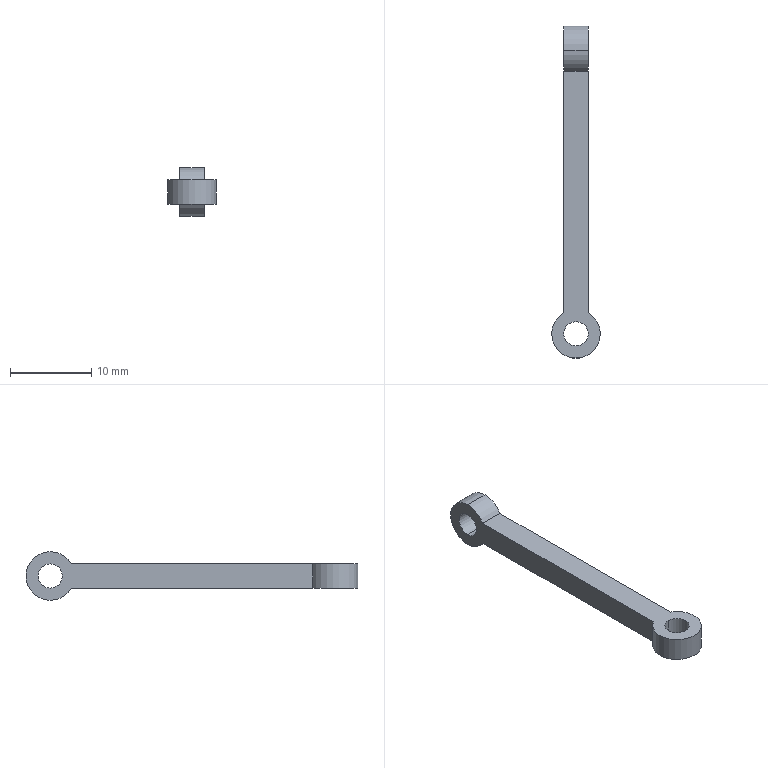Component | SolidWorks | 7-1 | 1 solid | 12 faces | box 6 x 41 x 6 mm | volume 391 mm3 | cylinder 8 | plane 4 | commonest cylinder face diameters 3 x4 6 x4
build123d program:
from build123d import *

# Parameters (mm, degrees)
BOSS_EXTRUDE1_DEPTH = 3
SKETCH2_R           = 1.5
CUT_EXTRUDE1_DEPTH  = 10
SKETCH4_W           = 5.598
SKETCH4_H           = 3
CUT_EXTRUDE2_DEPTH  = 4.5
SKETCH5_R           = 3
SKETCH5_R_2         = 1.5
BOSS_EXTRUDE2_DEPTH = 1.5


with BuildPart() as part:
    # Sketch1 → Boss-Extrude1 (new body)
    with BuildSketch(Plane.XY):
        with BuildLine():
            Line((32.402, 1.5), (2.598, 1.5))
            ThreePointArc((2.598, 1.5), (-3, 0), (2.598, -1.5))
            Line((2.598, -1.5), (32.402, -1.5))
            ThreePointArc((32.402, -1.5), (38, 0), (32.402, 1.5))
        make_face()
    extrude(amount=BOSS_EXTRUDE1_DEPTH)

    # Sketch2 → Cut-Extrude1 (cut)
    with BuildSketch(Plane.XY.offset(3)):
        Circle(SKETCH2_R)
        with Locations((35, 0)):
            Circle(SKETCH2_R)
    extrude(amount=-CUT_EXTRUDE1_DEPTH, mode=Mode.SUBTRACT)

    # Sketch4 → Cut-Extrude2 (cut, symmetric)
    with BuildSketch(Plane(origin=(0, 0, 0), x_dir=(1, 0, 0), z_dir=(0, 1, 0))):
        with Locations((-0.201, -1.5)):
            Rectangle(SKETCH4_W, SKETCH4_H)
    extrude(amount=CUT_EXTRUDE2_DEPTH, both=True, mode=Mode.SUBTRACT)

    # Sketch5 → Boss-Extrude2 (add, symmetric)
    with BuildSketch(Plane(origin=(0, 0, 0), x_dir=(1, 0, 0), z_dir=(0, 1, 0))):
        with Locations((0, -1.5)):
            Circle(SKETCH5_R)
        with Locations(Location((0, -1.5, 0), (0, 0, 270))):
            Circle(SKETCH5_R_2, mode=Mode.SUBTRACT)
    extrude(amount=BOSS_EXTRUDE2_DEPTH, both=True)


solid = part.part

# Placed as in the assembly
solid = solid.moved(Location((65.747, 70.686, -27.938), (0, 0, -90)))
STEP:
#1=COLOUR_RGB('',0.7922,0.8196,0.9333);
#2=FILL_AREA_STYLE_COLOUR('',#1);
#3=FILL_AREA_STYLE('',(#2));
#4=SURFACE_STYLE_FILL_AREA(#3);
#5=SURFACE_SIDE_STYLE('',(#4));
#6=SURFACE_STYLE_USAGE(.BOTH.,#5);
#7=PRESENTATION_STYLE_ASSIGNMENT((#6));
#8=CARTESIAN_POINT('',(2.648,2.783,-1.1));
#9=VERTEX_POINT('',#8);
#10=CARTESIAN_POINT('',(2.648,2.783,-0.9818));
#11=VERTEX_POINT('',#10);
#12=CARTESIAN_POINT('',(2.648,2.783,-1.041));
#13=DIRECTION('',(1.,-0.,0.));
#14=DIRECTION('',(0.,0.,1.));
#15=AXIS2_PLACEMENT_3D('',#12,#13,#14);
#16=CIRCLE('',#15,0.05906);
#17=EDGE_CURVE('',#9,#11,#16,.T.);
#18=ORIENTED_EDGE('',*,*,#17,.T.);
#19=CARTESIAN_POINT('',(2.529,2.783,-0.9818));
#20=VERTEX_POINT('',#19);
#21=CARTESIAN_POINT('',(2.648,2.783,-0.9818));
#22=DIRECTION('',(-1.,0.,-0.));
#23=VECTOR('',#22,39.37);
#24=LINE('',#21,#23);
#25=EDGE_CURVE('',#11,#20,#24,.T.);
#26=ORIENTED_EDGE('',*,*,#25,.T.);
#27=CARTESIAN_POINT('',(2.529,2.783,-1.1));
#28=VERTEX_POINT('',#27);
#29=CARTESIAN_POINT('',(2.529,2.783,-1.041));
#30=DIRECTION('',(1.,-0.,0.));
#31=DIRECTION('',(0.,0.,1.));
#32=AXIS2_PLACEMENT_3D('',#29,#30,#31);
#33=CIRCLE('',#32,0.05906);
#34=EDGE_CURVE('',#28,#20,#33,.T.);
#35=ORIENTED_EDGE('',*,*,#34,.F.);
#36=CARTESIAN_POINT('',(2.648,2.783,-1.1));
#37=DIRECTION('',(-1.,0.,-0.));
#38=VECTOR('',#37,39.37);
#39=LINE('',#36,#38);
#40=EDGE_CURVE('',#9,#28,#39,.T.);
#41=ORIENTED_EDGE('',*,*,#40,.F.);
#42=EDGE_LOOP('',(#18,#26,#35,#41));
#43=FACE_OUTER_BOUND('',#42,.T.);
#44=CARTESIAN_POINT('',(2.648,2.783,-1.041));
#45=DIRECTION('',(-1.,0.,-0.));
#46=DIRECTION('',(0.,0.,-1.));
#47=AXIS2_PLACEMENT_3D('',#44,#45,#46);
#48=CYLINDRICAL_SURFACE('',#47,0.05906);
#49=ADVANCED_FACE('',(#43),#48,.F.);
#50=CARTESIAN_POINT('',(2.648,2.783,-0.9228));
#51=VERTEX_POINT('',#50);
#52=CARTESIAN_POINT('',(2.648,2.681,-0.9818));
#53=VERTEX_POINT('',#52);
#54=CARTESIAN_POINT('',(2.648,2.783,-1.041));
#55=DIRECTION('',(1.,-0.,0.));
#56=DIRECTION('',(0.,0.,1.));
#57=AXIS2_PLACEMENT_3D('',#54,#55,#56);
#58=CIRCLE('',#57,0.1181);
#59=EDGE_CURVE('',#51,#53,#58,.T.);
#60=ORIENTED_EDGE('',*,*,#59,.F.);
#61=CARTESIAN_POINT('',(2.529,2.783,-0.9228));
#62=VERTEX_POINT('',#61);
#63=CARTESIAN_POINT('',(2.648,2.783,-0.9228));
#64=DIRECTION('',(-1.,0.,-0.));
#65=VECTOR('',#64,39.37);
#66=LINE('',#63,#65);
#67=EDGE_CURVE('',#51,#62,#66,.T.);
#68=ORIENTED_EDGE('',*,*,#67,.T.);
#69=CARTESIAN_POINT('',(2.529,2.681,-0.9818));
#70=VERTEX_POINT('',#69);
#71=CARTESIAN_POINT('',(2.529,2.783,-1.041));
#72=DIRECTION('',(1.,-0.,0.));
#73=DIRECTION('',(0.,0.,1.));
#74=AXIS2_PLACEMENT_3D('',#71,#72,#73);
#75=CIRCLE('',#74,0.1181);
#76=EDGE_CURVE('',#62,#70,#75,.T.);
#77=ORIENTED_EDGE('',*,*,#76,.T.);
#78=CARTESIAN_POINT('',(2.411,2.681,-0.9818));
#79=DIRECTION('',(1.,-0.,0.));
#80=VECTOR('',#79,39.37);
#81=LINE('',#78,#80);
#82=EDGE_CURVE('',#70,#53,#81,.T.);
#83=ORIENTED_EDGE('',*,*,#82,.T.);
#84=EDGE_LOOP('',(#60,#68,#77,#83));
#85=FACE_OUTER_BOUND('',#84,.T.);
#86=CARTESIAN_POINT('',(2.648,2.783,-1.041));
#87=DIRECTION('',(-1.,0.,-0.));
#88=DIRECTION('',(0.,0.,-1.));
#89=AXIS2_PLACEMENT_3D('',#86,#87,#88);
#90=CYLINDRICAL_SURFACE('',#89,0.1181);
#91=ADVANCED_FACE('',(#85),#90,.T.);
#92=ORIENTED_EDGE('',*,*,#67,.F.);
#93=CARTESIAN_POINT('',(2.648,2.783,-1.159));
#94=VERTEX_POINT('',#93);
#95=CARTESIAN_POINT('',(2.648,2.783,-1.041));
#96=DIRECTION('',(1.,-0.,0.));
#97=DIRECTION('',(0.,0.,1.));
#98=AXIS2_PLACEMENT_3D('',#95,#96,#97);
#99=CIRCLE('',#98,0.1181);
#100=EDGE_CURVE('',#94,#51,#99,.T.);
#101=ORIENTED_EDGE('',*,*,#100,.F.);
#102=CARTESIAN_POINT('',(2.529,2.783,-1.159));
#103=VERTEX_POINT('',#102);
#104=CARTESIAN_POINT('',(2.648,2.783,-1.159));
#105=DIRECTION('',(-1.,0.,-0.));
#106=VECTOR('',#105,39.37);
#107=LINE('',#104,#106);
#108=EDGE_CURVE('',#94,#103,#107,.T.);
#109=ORIENTED_EDGE('',*,*,#108,.T.);
#110=CARTESIAN_POINT('',(2.529,2.783,-1.041));
#111=DIRECTION('',(1.,-0.,0.));
#112=DIRECTION('',(0.,0.,1.));
#113=AXIS2_PLACEMENT_3D('',#110,#111,#112);
#114=CIRCLE('',#113,0.1181);
#115=EDGE_CURVE('',#103,#62,#114,.T.);
#116=ORIENTED_EDGE('',*,*,#115,.T.);
#117=EDGE_LOOP('',(#92,#101,#109,#116));
#118=FACE_OUTER_BOUND('',#117,.T.);
#119=CARTESIAN_POINT('',(2.648,2.783,-1.041));
#120=DIRECTION('',(-1.,0.,-0.));
#121=DIRECTION('',(0.,0.,-1.));
#122=AXIS2_PLACEMENT_3D('',#119,#120,#121);
#123=CYLINDRICAL_SURFACE('',#122,0.1181);
#124=ADVANCED_FACE('',(#118),#123,.T.);
#125=CARTESIAN_POINT('',(2.588,1.464,-1.1));
#126=VERTEX_POINT('',#125);
#127=CARTESIAN_POINT('',(2.588,1.346,-1.1));
#128=VERTEX_POINT('',#127);
#129=CARTESIAN_POINT('',(2.588,1.405,-1.1));
#130=DIRECTION('',(-0.,0.,1.));
#131=DIRECTION('',(0.,-1.,0.));
#132=AXIS2_PLACEMENT_3D('',#129,#130,#131);
#133=CIRCLE('',#132,0.05906);
#134=EDGE_CURVE('',#126,#128,#133,.T.);
#135=ORIENTED_EDGE('',*,*,#134,.F.);
#136=CARTESIAN_POINT('',(2.588,1.464,-0.9818));
#137=VERTEX_POINT('',#136);
#138=CARTESIAN_POINT('',(2.588,1.464,-1.376));
#139=DIRECTION('',(-0.,0.,1.));
#140=VECTOR('',#139,39.37);
#141=LINE('',#138,#140);
#142=EDGE_CURVE('',#126,#137,#141,.T.);
#143=ORIENTED_EDGE('',*,*,#142,.T.);
#144=CARTESIAN_POINT('',(2.588,1.346,-0.9818));
#145=VERTEX_POINT('',#144);
#146=CARTESIAN_POINT('',(2.588,1.405,-0.9818));
#147=DIRECTION('',(-0.,0.,1.));
#148=DIRECTION('',(0.,-1.,0.));
#149=AXIS2_PLACEMENT_3D('',#146,#147,#148);
#150=CIRCLE('',#149,0.05906);
#151=EDGE_CURVE('',#137,#145,#150,.T.);
#152=ORIENTED_EDGE('',*,*,#151,.T.);
#153=CARTESIAN_POINT('',(2.588,1.346,-1.376));
#154=DIRECTION('',(-0.,0.,1.));
#155=VECTOR('',#154,39.37);
#156=LINE('',#153,#155);
#157=EDGE_CURVE('',#128,#145,#156,.T.);
#158=ORIENTED_EDGE('',*,*,#157,.F.);
#159=EDGE_LOOP('',(#135,#143,#152,#158));
#160=FACE_OUTER_BOUND('',#159,.T.);
#161=CARTESIAN_POINT('',(2.588,1.405,-1.376));
#162=DIRECTION('',(-0.,0.,1.));
#163=DIRECTION('',(0.,-1.,0.));
#164=AXIS2_PLACEMENT_3D('',#161,#162,#163);
#165=CYLINDRICAL_SURFACE('',#164,0.05906);
#166=ADVANCED_FACE('',(#160),#165,.F.);
#167=CARTESIAN_POINT('',(2.529,2.681,-1.1));
#168=VERTEX_POINT('',#167);
#169=CARTESIAN_POINT('',(2.529,2.783,-1.041));
#170=DIRECTION('',(1.,-0.,0.));
#171=DIRECTION('',(0.,0.,1.));
#172=AXIS2_PLACEMENT_3D('',#169,#170,#171);
#173=CIRCLE('',#172,0.1181);
#174=EDGE_CURVE('',#168,#103,#173,.T.);
#175=ORIENTED_EDGE('',*,*,#174,.F.);
#176=CARTESIAN_POINT('',(2.529,1.507,-1.1));
#177=VERTEX_POINT('',#176);
#178=CARTESIAN_POINT('',(2.529,2.783,-1.1));
#179=DIRECTION('',(-0.,-1.,0.));
#180=VECTOR('',#179,39.37);
#181=LINE('',#178,#180);
#182=EDGE_CURVE('',#168,#177,#181,.T.);
#183=ORIENTED_EDGE('',*,*,#182,.T.);
#184=CARTESIAN_POINT('',(2.529,1.507,-0.9818));
#185=VERTEX_POINT('',#184);
#186=CARTESIAN_POINT('',(2.529,1.507,-0.9818));
#187=DIRECTION('',(0.,-0.,-1.));
#188=VECTOR('',#187,39.37);
#189=LINE('',#186,#188);
#190=EDGE_CURVE('',#185,#177,#189,.T.);
#191=ORIENTED_EDGE('',*,*,#190,.F.);
#192=CARTESIAN_POINT('',(2.529,2.783,-0.9818));
#193=DIRECTION('',(-0.,-1.,0.));
#194=VECTOR('',#193,39.37);
#195=LINE('',#192,#194);
#196=EDGE_CURVE('',#70,#185,#195,.T.);
#197=ORIENTED_EDGE('',*,*,#196,.F.);
#198=ORIENTED_EDGE('',*,*,#76,.F.);
#199=ORIENTED_EDGE('',*,*,#115,.F.);
#200=EDGE_LOOP('',(#175,#183,#191,#197,#198,#199));
#201=FACE_OUTER_BOUND('',#200,.T.);
#202=ORIENTED_EDGE('',*,*,#34,.T.);
#203=CARTESIAN_POINT('',(2.529,2.783,-1.041));
#204=DIRECTION('',(1.,-0.,0.));
#205=DIRECTION('',(0.,0.,1.));
#206=AXIS2_PLACEMENT_3D('',#203,#204,#205);
#207=CIRCLE('',#206,0.05906);
#208=EDGE_CURVE('',#20,#28,#207,.T.);
#209=ORIENTED_EDGE('',*,*,#208,.T.);
#210=EDGE_LOOP('',(#202,#209));
#211=FACE_BOUND('',#210,.T.);
#212=CARTESIAN_POINT('',(2.529,2.783,-0.9818));
#213=DIRECTION('',(1.,-0.,0.));
#214=DIRECTION('',(-0.,0.,1.));
#215=AXIS2_PLACEMENT_3D('',#212,#213,#214);
#216=PLANE('',#215);
#217=ADVANCED_FACE('',(#201,#211),#216,.F.);
#218=CARTESIAN_POINT('',(2.648,1.507,-1.1));
#219=VERTEX_POINT('',#218);
#220=CARTESIAN_POINT('',(2.588,1.405,-1.1));
#221=DIRECTION('',(-0.,0.,1.));
#222=DIRECTION('',(0.,-1.,0.));
#223=AXIS2_PLACEMENT_3D('',#220,#221,#222);
#224=CIRCLE('',#223,0.1181);
#225=EDGE_CURVE('',#177,#219,#224,.T.);
#226=ORIENTED_EDGE('',*,*,#225,.T.);
#227=CARTESIAN_POINT('',(2.648,1.507,-0.9818));
#228=VERTEX_POINT('',#227);
#229=CARTESIAN_POINT('',(2.648,1.507,-0.9818));
#230=DIRECTION('',(0.,-0.,-1.));
#231=VECTOR('',#230,39.37);
#232=LINE('',#229,#231);
#233=EDGE_CURVE('',#228,#219,#232,.T.);
#234=ORIENTED_EDGE('',*,*,#233,.F.);
#235=CARTESIAN_POINT('',(2.588,1.405,-0.9818));
#236=DIRECTION('',(-0.,0.,1.));
#237=DIRECTION('',(0.,-1.,0.));
#238=AXIS2_PLACEMENT_3D('',#235,#236,#237);
#239=CIRCLE('',#238,0.1181);
#240=EDGE_CURVE('',#185,#228,#239,.T.);
#241=ORIENTED_EDGE('',*,*,#240,.F.);
#242=ORIENTED_EDGE('',*,*,#190,.T.);
#243=EDGE_LOOP('',(#226,#234,#241,#242));
#244=FACE_OUTER_BOUND('',#243,.T.);
#245=CARTESIAN_POINT('',(2.588,1.405,-0.9818));
#246=DIRECTION('',(0.,-0.,-1.));
#247=DIRECTION('',(0.,1.,0.));
#248=AXIS2_PLACEMENT_3D('',#245,#246,#247);
#249=CYLINDRICAL_SURFACE('',#248,0.1181);
#250=ADVANCED_FACE('',(#244),#249,.T.);
#251=CARTESIAN_POINT('',(2.648,2.681,-1.1));
#252=VERTEX_POINT('',#251);
#253=CARTESIAN_POINT('',(2.648,2.783,-1.041));
#254=DIRECTION('',(1.,-0.,0.));
#255=DIRECTION('',(0.,0.,1.));
#256=AXIS2_PLACEMENT_3D('',#253,#254,#255);
#257=CIRCLE('',#256,0.1181);
#258=EDGE_CURVE('',#252,#94,#257,.T.);
#259=ORIENTED_EDGE('',*,*,#258,.T.);
#260=ORIENTED_EDGE('',*,*,#100,.T.);
#261=ORIENTED_EDGE('',*,*,#59,.T.);
#262=CARTESIAN_POINT('',(2.648,2.783,-0.9818));
#263=DIRECTION('',(-0.,-1.,0.));
#264=VECTOR('',#263,39.37);
#265=LINE('',#262,#264);
#266=EDGE_CURVE('',#53,#228,#265,.T.);
#267=ORIENTED_EDGE('',*,*,#266,.T.);
#268=ORIENTED_EDGE('',*,*,#233,.T.);
#269=CARTESIAN_POINT('',(2.648,2.783,-1.1));
#270=DIRECTION('',(-0.,-1.,0.));
#271=VECTOR('',#270,39.37);
#272=LINE('',#269,#271);
#273=EDGE_CURVE('',#252,#219,#272,.T.);
#274=ORIENTED_EDGE('',*,*,#273,.F.);
#275=EDGE_LOOP('',(#259,#260,#261,#267,#268,#274));
#276=FACE_OUTER_BOUND('',#275,.T.);
#277=ORIENTED_EDGE('',*,*,#17,.F.);
#278=CARTESIAN_POINT('',(2.648,2.783,-1.041));
#279=DIRECTION('',(1.,-0.,0.));
#280=DIRECTION('',(0.,0.,1.));
#281=AXIS2_PLACEMENT_3D('',#278,#279,#280);
#282=CIRCLE('',#281,0.05906);
#283=EDGE_CURVE('',#11,#9,#282,.T.);
#284=ORIENTED_EDGE('',*,*,#283,.F.);
#285=EDGE_LOOP('',(#277,#284));
#286=FACE_BOUND('',#285,.T.);
#287=CARTESIAN_POINT('',(2.648,2.783,-0.9818));
#288=DIRECTION('',(1.,-0.,0.));
#289=DIRECTION('',(-0.,0.,1.));
#290=AXIS2_PLACEMENT_3D('',#287,#288,#289);
#291=PLANE('',#290);
#292=ADVANCED_FACE('',(#276,#286),#291,.T.);
#293=ORIENTED_EDGE('',*,*,#82,.F.);
#294=ORIENTED_EDGE('',*,*,#196,.T.);
#295=ORIENTED_EDGE('',*,*,#240,.T.);
#296=ORIENTED_EDGE('',*,*,#266,.F.);
#297=EDGE_LOOP('',(#293,#294,#295,#296));
#298=FACE_OUTER_BOUND('',#297,.T.);
#299=CARTESIAN_POINT('',(2.588,1.405,-0.9818));
#300=DIRECTION('',(-0.,0.,1.));
#301=DIRECTION('',(0.,-1.,0.));
#302=AXIS2_PLACEMENT_3D('',#299,#300,#301);
#303=CIRCLE('',#302,0.05906);
#304=EDGE_CURVE('',#145,#137,#303,.T.);
#305=ORIENTED_EDGE('',*,*,#304,.F.);
#306=ORIENTED_EDGE('',*,*,#151,.F.);
#307=EDGE_LOOP('',(#305,#306));
#308=FACE_BOUND('',#307,.T.);
#309=CARTESIAN_POINT('',(2.588,2.783,-0.9818));
#310=DIRECTION('',(-0.,0.,1.));
#311=DIRECTION('',(-0.,-1.,0.));
#312=AXIS2_PLACEMENT_3D('',#309,#310,#311);
#313=PLANE('',#312);
#314=ADVANCED_FACE('',(#298,#308),#313,.T.);
#315=CARTESIAN_POINT('',(2.588,1.405,-1.1));
#316=DIRECTION('',(-0.,0.,1.));
#317=DIRECTION('',(0.,-1.,0.));
#318=AXIS2_PLACEMENT_3D('',#315,#316,#317);
#319=CIRCLE('',#318,0.05906);
#320=EDGE_CURVE('',#128,#126,#319,.T.);
#321=ORIENTED_EDGE('',*,*,#320,.T.);
#322=ORIENTED_EDGE('',*,*,#134,.T.);
#323=EDGE_LOOP('',(#321,#322));
#324=FACE_BOUND('',#323,.T.);
#325=ORIENTED_EDGE('',*,*,#182,.F.);
#326=CARTESIAN_POINT('',(2.411,2.681,-1.1));
#327=DIRECTION('',(1.,-0.,0.));
#328=VECTOR('',#327,39.37);
#329=LINE('',#326,#328);
#330=EDGE_CURVE('',#168,#252,#329,.T.);
#331=ORIENTED_EDGE('',*,*,#330,.T.);
#332=ORIENTED_EDGE('',*,*,#273,.T.);
#333=ORIENTED_EDGE('',*,*,#225,.F.);
#334=EDGE_LOOP('',(#325,#331,#332,#333));
#335=FACE_OUTER_BOUND('',#334,.T.);
#336=CARTESIAN_POINT('',(2.588,2.783,-1.1));
#337=DIRECTION('',(-0.,0.,1.));
#338=DIRECTION('',(-0.,-1.,0.));
#339=AXIS2_PLACEMENT_3D('',#336,#337,#338);
#340=PLANE('',#339);
#341=ADVANCED_FACE('',(#324,#335),#340,.F.);
#342=ORIENTED_EDGE('',*,*,#142,.F.);
#343=ORIENTED_EDGE('',*,*,#320,.F.);
#344=ORIENTED_EDGE('',*,*,#157,.T.);
#345=ORIENTED_EDGE('',*,*,#304,.T.);
#346=EDGE_LOOP('',(#342,#343,#344,#345));
#347=FACE_OUTER_BOUND('',#346,.T.);
#348=CARTESIAN_POINT('',(2.588,1.405,-1.376));
#349=DIRECTION('',(-0.,0.,1.));
#350=DIRECTION('',(0.,-1.,0.));
#351=AXIS2_PLACEMENT_3D('',#348,#349,#350);
#352=CYLINDRICAL_SURFACE('',#351,0.05906);
#353=ADVANCED_FACE('',(#347),#352,.F.);
#354=ORIENTED_EDGE('',*,*,#108,.F.);
#355=ORIENTED_EDGE('',*,*,#258,.F.);
#356=ORIENTED_EDGE('',*,*,#330,.F.);
#357=ORIENTED_EDGE('',*,*,#174,.T.);
#358=EDGE_LOOP('',(#354,#355,#356,#357));
#359=FACE_OUTER_BOUND('',#358,.T.);
#360=CARTESIAN_POINT('',(2.648,2.783,-1.041));
#361=DIRECTION('',(-1.,0.,-0.));
#362=DIRECTION('',(0.,0.,-1.));
#363=AXIS2_PLACEMENT_3D('',#360,#361,#362);
#364=CYLINDRICAL_SURFACE('',#363,0.1181);
#365=ADVANCED_FACE('',(#359),#364,.T.);
#366=ORIENTED_EDGE('',*,*,#25,.F.);
#367=ORIENTED_EDGE('',*,*,#283,.T.);
#368=ORIENTED_EDGE('',*,*,#40,.T.);
#369=ORIENTED_EDGE('',*,*,#208,.F.);
#370=EDGE_LOOP('',(#366,#367,#368,#369));
#371=FACE_OUTER_BOUND('',#370,.T.);
#372=CARTESIAN_POINT('',(2.648,2.783,-1.041));
#373=DIRECTION('',(-1.,0.,-0.));
#374=DIRECTION('',(0.,0.,-1.));
#375=AXIS2_PLACEMENT_3D('',#372,#373,#374);
#376=CYLINDRICAL_SURFACE('',#375,0.05906);
#377=ADVANCED_FACE('',(#371),#376,.F.);
#378=CLOSED_SHELL('',(#49,#91,#124,#166,#217,#250,#292,#314,#341,#353,#365,#377));
#379=MANIFOLD_SOLID_BREP('',#378);
#380=STYLED_ITEM('',(#7),#379);
#381=PRESENTATION_LAYER_ASSIGNMENT('','',(#380));
#382=(LENGTH_UNIT()NAMED_UNIT(*)SI_UNIT($,.METRE.));
#383=LENGTH_MEASURE_WITH_UNIT(LENGTH_MEASURE(0.0254),#382);
#384=DIMENSIONAL_EXPONENTS(1.,0.,0.,0.,0.,0.,0.);
#385=(CONVERSION_BASED_UNIT('',#383)LENGTH_UNIT()NAMED_UNIT(#384));
#386=UNCERTAINTY_MEASURE_WITH_UNIT(LENGTH_MEASURE(0.00001),#385,'','');
#387=(NAMED_UNIT(*)PLANE_ANGLE_UNIT()SI_UNIT($,.RADIAN.));
#388=(NAMED_UNIT(*)SI_UNIT($,.STERADIAN.)SOLID_ANGLE_UNIT());
#389=(GEOMETRIC_REPRESENTATION_CONTEXT(3)GLOBAL_UNCERTAINTY_ASSIGNED_CONTEXT((#386))GLOBAL_UNIT_ASSIGNED_CONTEXT((#385,#387,#388))REPRESENTATION_CONTEXT('',''));
#390=MECHANICAL_DESIGN_GEOMETRIC_PRESENTATION_REPRESENTATION('',(#380),#389);
#391=CARTESIAN_POINT('',(0.,0.,0.));
#392=DIRECTION('',(0.,0.,1.));
#393=DIRECTION('',(1.,0.,0.));
#394=AXIS2_PLACEMENT_3D('',#391,#392,#393);
#395=(LENGTH_UNIT()NAMED_UNIT(*)SI_UNIT($,.METRE.));
#396=LENGTH_MEASURE_WITH_UNIT(LENGTH_MEASURE(0.0254),#395);
#397=DIMENSIONAL_EXPONENTS(1.,0.,0.,0.,0.,0.,0.);
#398=(CONVERSION_BASED_UNIT('',#396)LENGTH_UNIT()NAMED_UNIT(#397));
#399=UNCERTAINTY_MEASURE_WITH_UNIT(LENGTH_MEASURE(0.00001),#398,'','');
#400=(NAMED_UNIT(*)PLANE_ANGLE_UNIT()SI_UNIT($,.RADIAN.));
#401=(NAMED_UNIT(*)SI_UNIT($,.STERADIAN.)SOLID_ANGLE_UNIT());
#402=(GEOMETRIC_REPRESENTATION_CONTEXT(3)GLOBAL_UNCERTAINTY_ASSIGNED_CONTEXT((#399))GLOBAL_UNIT_ASSIGNED_CONTEXT((#398,#400,#401))REPRESENTATION_CONTEXT('',''));
#403=ADVANCED_BREP_SHAPE_REPRESENTATION('',(#379,#394),#402);